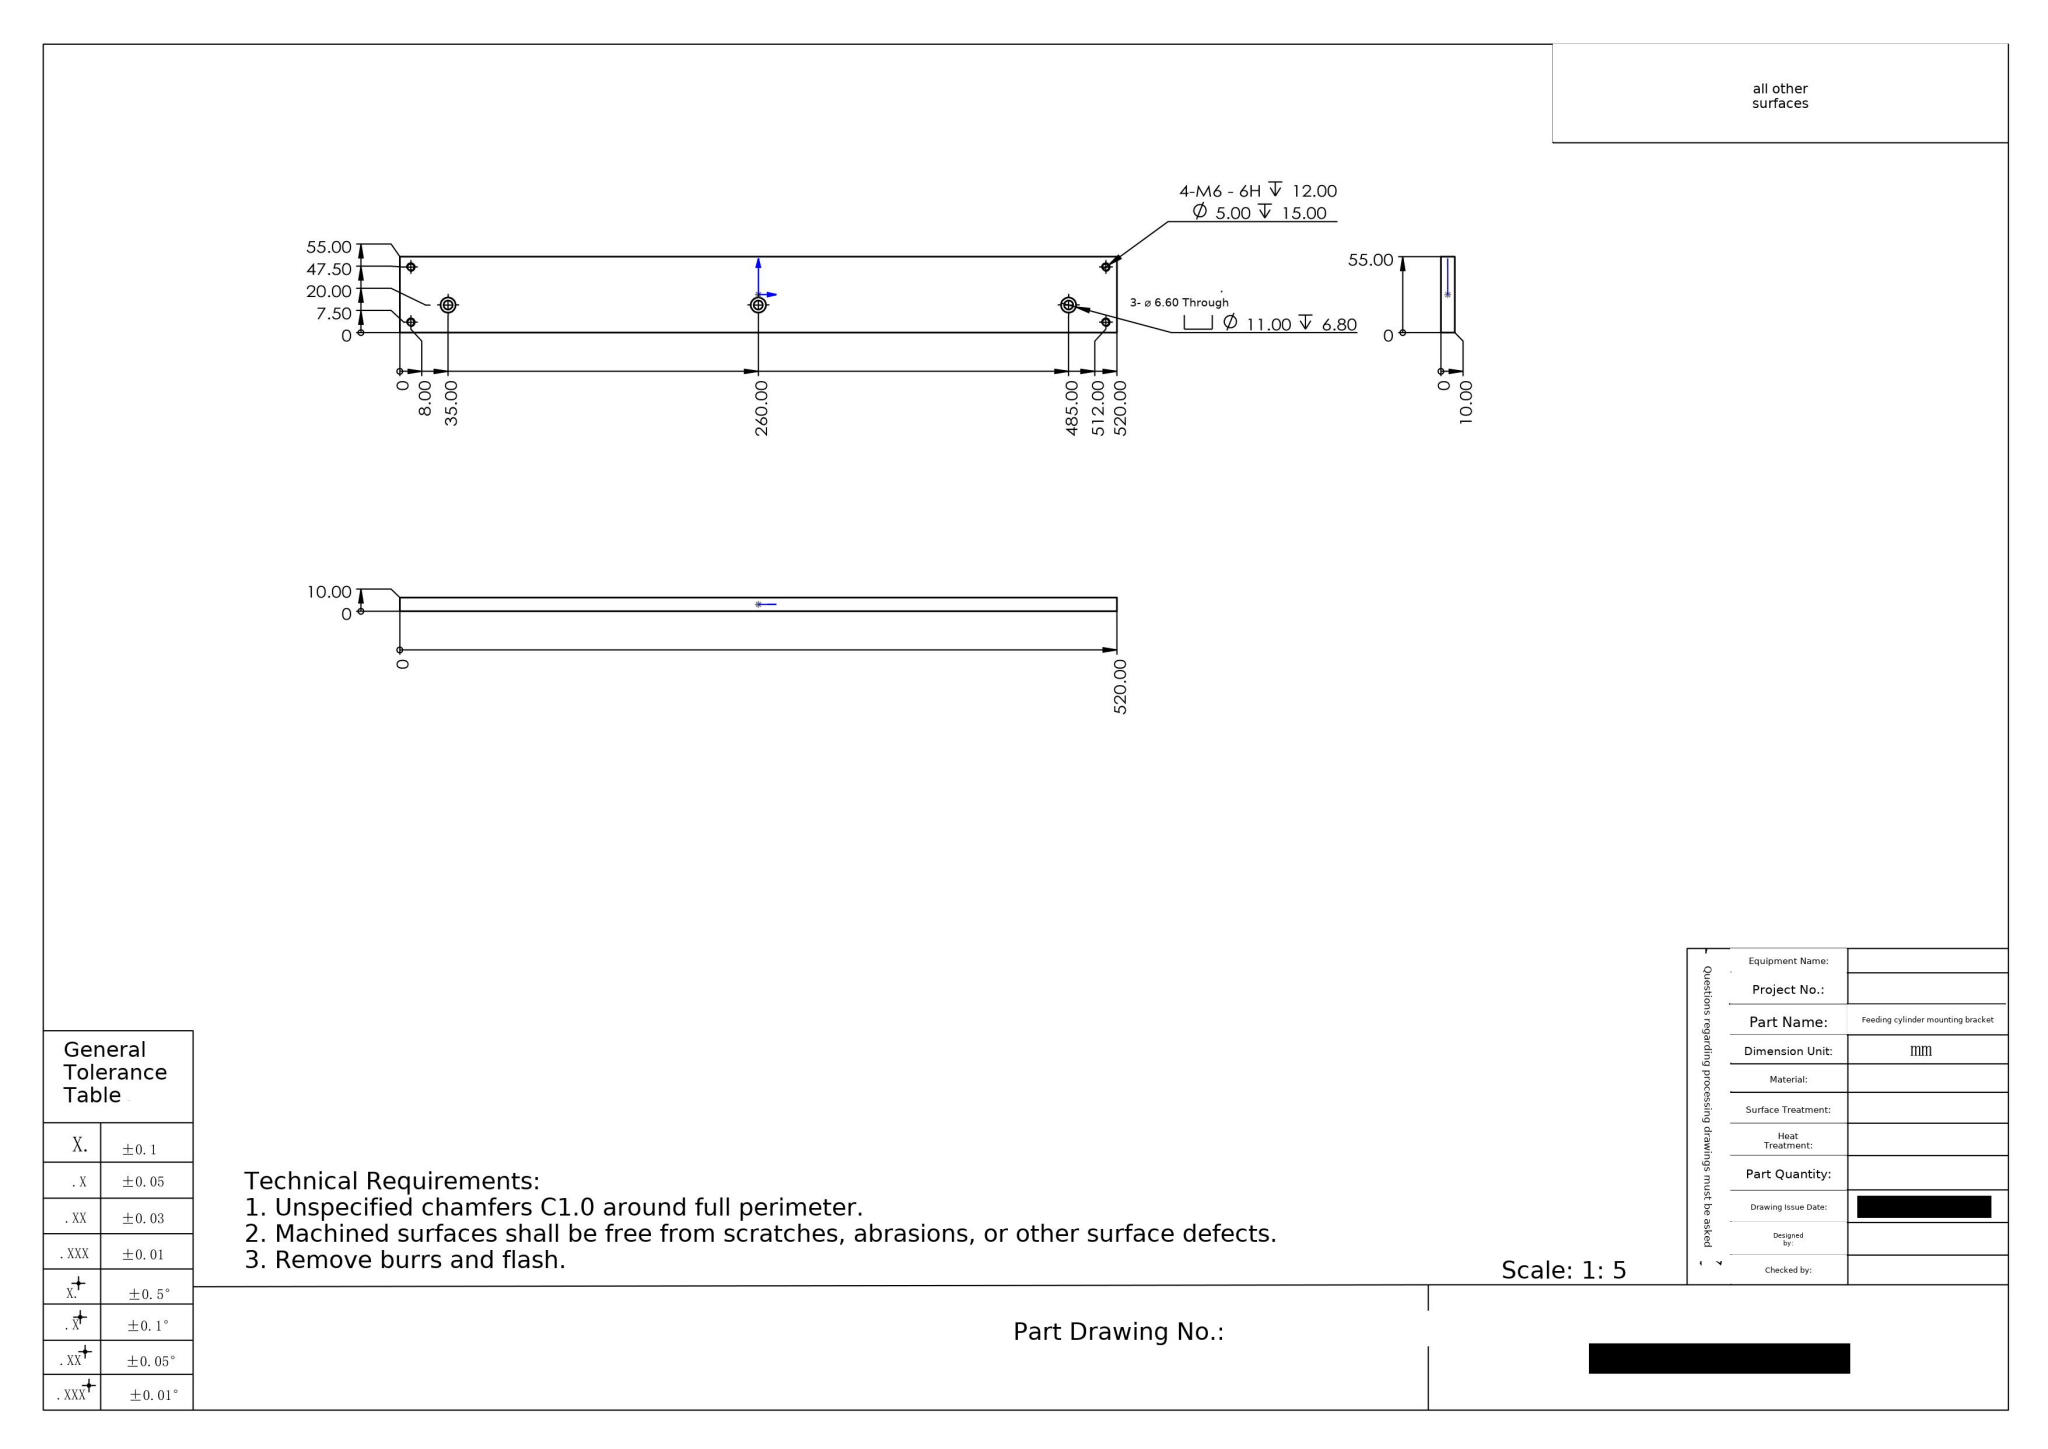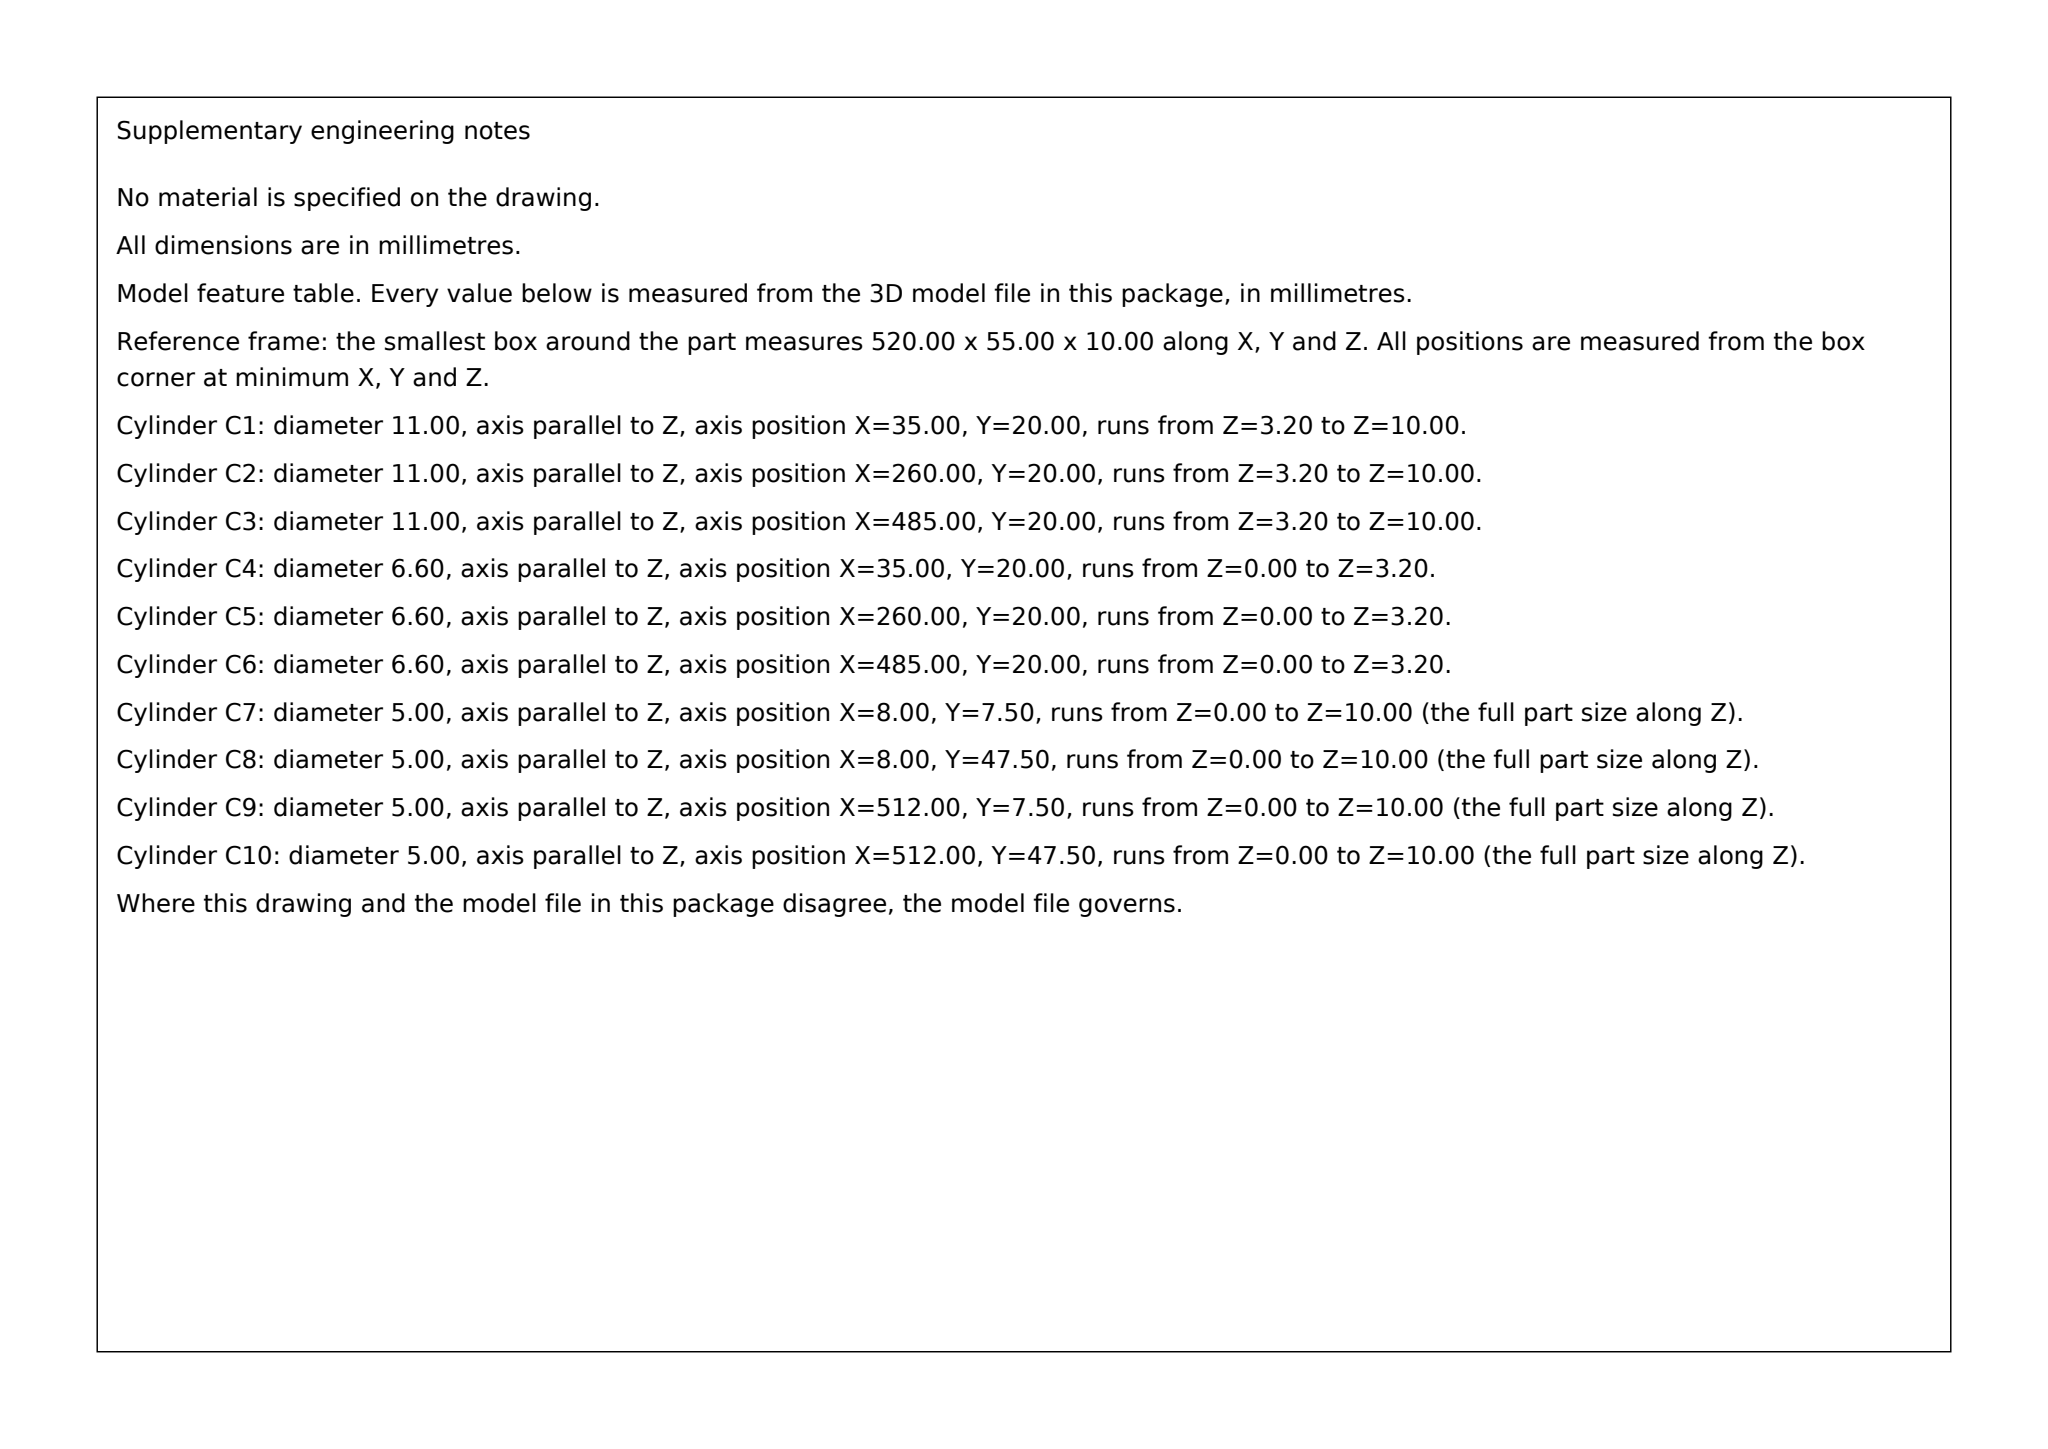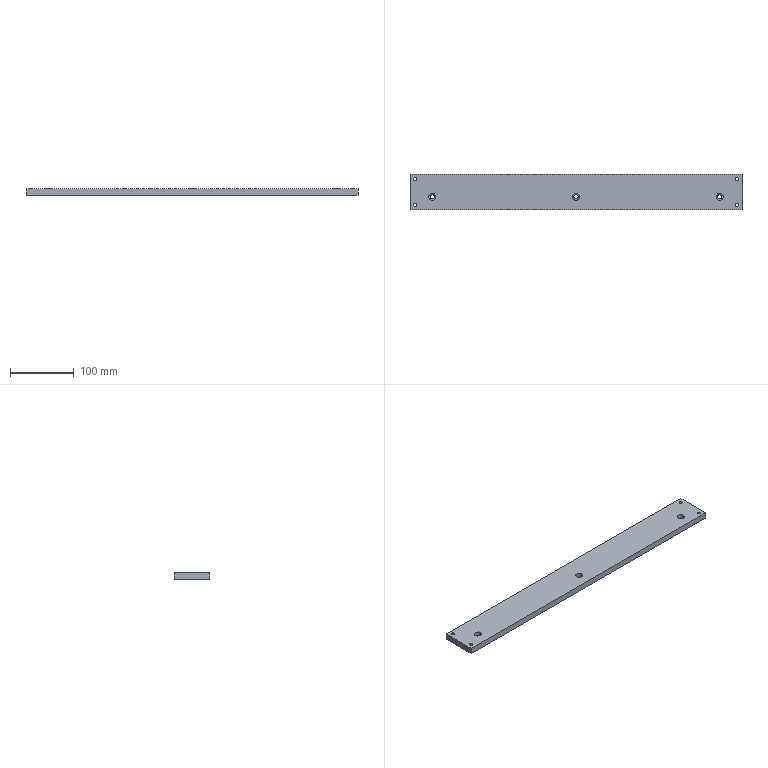Part | SolidWorks | mm | 1 solid | 29 faces | box 520 x 55 x 10 mm | volume 282947 mm3 | cylinder 20 | plane 9 | commonest cylinder face diameters 5 x8 11 x6 6.6 x6
build123d program:
from build123d import *

# Parameters (mm, degrees)
SKETCH1_W                                            = 520
SKETCH1_H                                            = 55
BOSS_EXTRUDE1_DEPTH                                  = 5
M6_TAPPED_HOLE1_D                                    = 5
M6_TAPPED_HOLE1_DEPTH                                = 15
M6_TAPPED_HOLE1_TIP                                  = 1.502
HOLE_SIZE_ACCORDING_TO_THE_TYPE_OF_HEXAG_D           = 6.6
HOLE_SIZE_ACCORDING_TO_THE_TYPE_OF_HEXAG_CBORE_D     = 11
HOLE_SIZE_ACCORDING_TO_THE_TYPE_OF_HEXAG_CBORE_DEPTH = 6.8


with BuildPart() as part:
    # Sketch1 → Boss-Extrude1 (new, symmetric)
    with BuildSketch(Plane.XY):
        Rectangle(SKETCH1_W, SKETCH1_H)
    extrude(amount=BOSS_EXTRUDE1_DEPTH, both=True)

    # M6 Tapped Hole1
    with Locations(Plane.XY.offset(5)):
        with Locations((252, 20), (252, -20), (-252, 20), (-252, -20)):
            Hole(M6_TAPPED_HOLE1_D / 2, depth=M6_TAPPED_HOLE1_DEPTH)
            with Locations((0, 0, -(M6_TAPPED_HOLE1_DEPTH + M6_TAPPED_HOLE1_TIP / 2))):  # 118° drill point
                Cone(0, M6_TAPPED_HOLE1_D / 2, M6_TAPPED_HOLE1_TIP, mode=Mode.SUBTRACT)

    # Hole size according to the type of hexag (through all)
    with Locations(Plane.XY.offset(5)):
        with Locations((-225, -7.5), (0, -7.5), (225, -7.5)):
            CounterBoreHole(HOLE_SIZE_ACCORDING_TO_THE_TYPE_OF_HEXAG_D / 2, HOLE_SIZE_ACCORDING_TO_THE_TYPE_OF_HEXAG_CBORE_D / 2, HOLE_SIZE_ACCORDING_TO_THE_TYPE_OF_HEXAG_CBORE_DEPTH)


solid = part.part